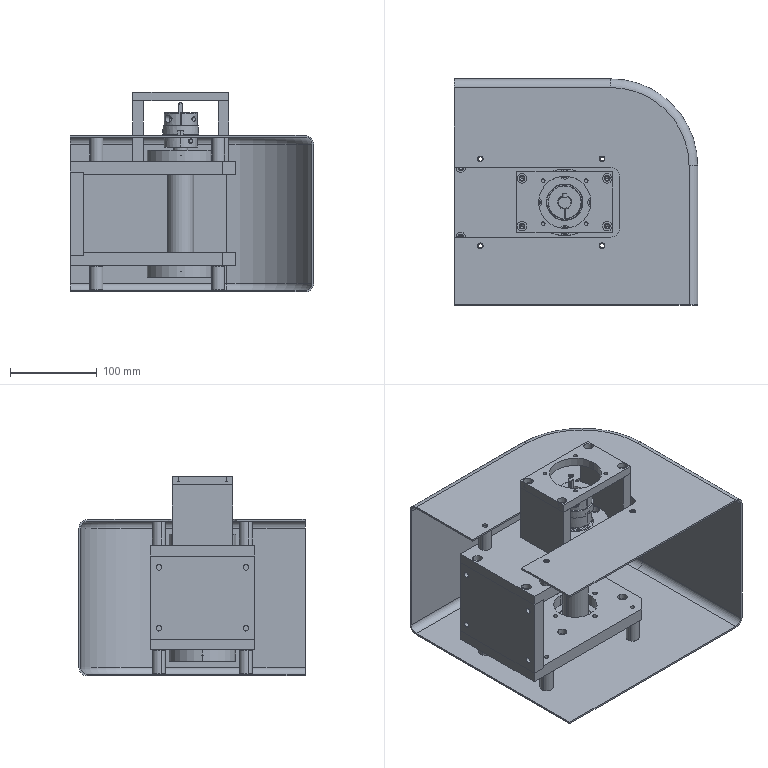Assembly | SolidWorks | mm | 30 component files | 30 solids | 814 faces | box 280 x 260 x 230 mm | volume 1605857 mm3 | cylinder 379 | plane 244 | cone 161 | torus 30 | commonest cylinder face diameters 5 x73 11 x56 6.6 x40 6.5 x32 6.647 x16 15 x16 16 x15 42 x12
Bill of materials:
10X8X50ParallelKey | 1 | AISI 1045 Steel, cold drawn | Flat bar with fully rounded (semicircular) ends, giving an obround outline, with small rounded edges all round.
17x5x5ParallelKey | 1 | AISI 1045 Steel, cold drawn | Thick obround prism (two parallel flat sides, semicircular ends) with chamfered edges on both faces.
25x5x5ParallelKey | 1 | AISI 1045 Steel, cold drawn | Slender obround prism with chamfered perimeter edges. Similar to the previous part but narrower relative to its length.
bearingB6905ZZ | 2 | AISI 1045 Steel, cold drawn | Plain annular ring (flat washer-like cylinder with a central through-bore). The top face shows thin concentric circular lines near the outer and inner edges.
housing_BGRRB6905ZZ | 2 | AISI 1045 Steel, cold drawn | Circular flange disc with a large central bore, four through-holes equally spaced on a bolt circle, and a shorter, smaller-diameter spigot/step on one face.
RRING42 | 2 | AISI 1045 Steel, cold drawn | Thin, flat, split ring with an open gap. Both ends have inward-projecting lugs, each with a small round hole.
M5 | 2 | AISI 1045 Steel, cold drawn | Headed cylindrical pin/screw-like body: a short, larger-diameter cylindrical head with a chamfered outer edge, and a longer smaller-diameter plain cylindrical shank with a chamfered tip.
MCOCG_spacer38 | 1 | AISI 1045 Steel, cold drawn | Thick annular disc with a central through-hole and a straight rectangular slot running across each face. The slots appear to sit at different angular positions, and a small notch is cut at the bore edge.
MCOCGXK3816 | 2 | AISI 1045 Steel, cold drawn | Split-type collar: a cylindrical ring with a central bore that has a rectangular keyway, a narrow radial slit through one side, transverse holes through the body, and a rectangular tab projecting axially from one face.
WT-FLD-EJG-1212-00-019 | 1 | AISI 1045 Steel, cold drawn | Flat rectangular plate with a large central circular through-opening, four larger corner holes, and four smaller holes arranged around the central opening.
WT-FLD-EJG-1212-00-020 | 2 | AISI 1045 Steel, cold drawn | Rectangular block/thick plate with plain large faces. Two round holes are drilled into one narrow edge face near each end.
WT-FLD-EJG-1212-00-006 | 2 | AISI 1045 Steel, cold drawn | Rectangular plate with two chamfered corners at one end. It has a large round through-opening offset toward the chamfered end, surrounded by four small holes at 90 degrees, several additional hole patterns, and a stepped edge (rabbet) on one side.
WT-FLD-EJG-1212-00-007 | 1 | AISI 1045 Steel, cold drawn | Thick rectangular plate block with four through holes near the corners of the large face and two small holes in one narrow edge face.
WT-FLD-EJG-1212-00-008 | 1 | AISI 1045 Steel, cold drawn | Stepped cylindrical shaft with a long main body, reduced-diameter steps at both ends, and a keyway slot on the smallest end journal.
WT-FLD-EJG-1212-00-023 | 1 | AISI 1045 Steel, cold drawn | Thin bent sheet part with a C-shaped cross-section: a top flange and a bottom flange joined by a vertical wall that wraps around one large-radius rounded corner in plan view.
WT-FLD-EJG-1212-00-024 | 8 | AISI 1045 Steel, cold drawn | Plain cylindrical tube or spacer with a central through bore and chamfered outer end edges.
Mates:
1. coincident | WT-FLD-EJG-1212-00-006-1 face at (-127, 0, 48) dir (0, 0, -1) | WT-FLD-EJG-1212-00-007-1 face at (-112, -60, 48) dir (0, 0, 1)
2. coincident | WT-FLD-EJG-1212-00-006-1 face at (-127, 0, 60) dir (0, 0, 1) | BGRRB6905ZZ-1/housing_BGRRB6905ZZ-1 face at (0, 0, 60) dir (0, 0, -1)
3. concentric | WT-FLD-EJG-1212-00-006-1 face at (0, 0, 45) dir (0, 0, 1) r 25 | BGRRB6905ZZ-1/housing_BGRRB6905ZZ-1 face at (0, 0, 60) dir (0, 0, -1) r 25
4. coincident | WT-FLD-EJG-1212-00-008-1 face at (0, 10, -25) dir (0, 1, 0) | 10X8X50ParallelKey-1 face at (0, 10, -25) dir (0, -1, 0)
5. concentric | WT-FLD-EJG-1212-00-008-1 face at (0, 15, 25) dir (0, -1, 0) r 5 | 10X8X50ParallelKey-1 face at (0, 10, 25) dir (0, 1, 0) r 5
6. concentric | WT-FLD-EJG-1212-00-008-1 face at (0, 15, -25) dir (0, -1, 0) r 5 | 10X8X50ParallelKey-1 face at (0, 10, -25) dir (0, 1, 0) r 5
7. concentric | WT-FLD-EJG-1212-00-008-1 face at (0, 0, -70) dir (0, 0, -1) r 15 | assembly face at (0, 0, 132) dir (0, 0, -1) r 8
8. parallel | WT-FLD-EJG-1212-00-006-1 face at (63, 60, 45) dir (0, 1, 0) | ServoDriveMotorModule-1/WT-FLD-EJG-1212-00-019-1 face at (-55, 35, 140) dir (0, 1, 0)
9. coincident | WT-FLD-EJG-1212-00-006-1 face at (-127, 0, 60) dir (0, 0, 1) | ServoDriveMotorModule-1/WT-FLD-EJG-1212-00-020-1 face at (-49, 0, 60) dir (0, 0, -1)
10. coincident | WT-FLD-EJG-1212-00-008-1 face at (0, 5, 75) dir (0, 1, 0) | 17x5x5ParallelKey-1 face at (0, 5, 87) dir (0, -1, 0)
11. concentric | WT-FLD-EJG-1212-00-008-1 face at (0, 15, 75) dir (0, -1, 0) r 2.5 | 17x5x5ParallelKey-1 face at (0, 10, 75) dir (0, -1, 0) r 2.5
12. coincident | WT-FLD-EJG-1212-00-008-1 face at (2.5, 15, 75) dir (-1, 0, 0) | 17x5x5ParallelKey-1 face at (2.5, 10, 87) dir (1, 0, 0)
13. coincident | assembly face at (2.5, 5, 103) dir (0, 1, 0) | 25x5x5ParallelKey-1 face at (0, 5, 105.5) dir (0, -1, 0)
14. concentric | assembly face at (0, 5.693, 125.5) dir (0, 1, 0) r 2.5 | 25x5x5ParallelKey-1 face at (0, 5, 125.5) dir (0, 1, 0) r 2.5
15. coincident | assembly face at (2.5, 7.599, 103) dir (-1, 0, 0) | 25x5x5ParallelKey-1 face at (2.5, 5, 105.5) dir (1, 0, 0)
16. parallel | WT-FLD-EJG-1212-00-006-1 plane at (-127, 0, 60) dir (1, 0, 0) | BGRRB6905ZZ-1 plane at (0, 0, 58) dir (-1, 0, 0)
17. concentric | WT-FLD-EJG-1212-00-006-1 face at (-119.5, 40, 60) dir (0, 0, 1) r 3.3 | WT-FLD-EJG-1212-00-007-1 face at (-119.5, 40, 48) dir (0, 0, 1) r 2.5
18. concentric | WT-FLD-EJG-1212-00-006-1 face at (-119.5, -40, 60) dir (0, 0, 1) r 3.3 | WT-FLD-EJG-1212-00-007-1 face at (-119.5, -40, 48) dir (0, 0, 1) r 2.5
19. coincident | WT-FLD-EJG-1212-00-007-1 face at (-127, 0, 0) dir (-1, 0, 0) | WT-FLD-EJG-1212-00-023-1 face at (-127, -118, -90) dir (-1, 0, 0)
20. coincident | WT-FLD-EJG-1212-00-023-1 plane at (-127, -118, 0) dir (0, 0, -1) | assembly plane at (0, 0, 0) dir (0, 0, 1)
21. distance | WT-FLD-EJG-1212-00-006-2 face at (63, 60, -45) dir (0, 1, 0) | WT-FLD-EJG-1212-00-023-1 face at (-127, 140, -90) dir (0, -1, 0)
22. coincident | WT-FLD-EJG-1212-00-006-1 face at (-127, 0, 60) dir (0, 0, 1) | WT-FLD-EJG-1212-00-024-1 face at (-97, -50, 60) dir (0, 0, -1)
23. concentric | WT-FLD-EJG-1212-00-006-1 face at (-97, -50, 60) dir (0, 0, 1) r 2.5 | WT-FLD-EJG-1212-00-024-1 face at (-97, -50, 60) dir (0, 0, -1) r 3.25
24. distance | bearingB6905ZZ-1 plane at (2, 0, 0) dir (1, 0, 0) | housing_BGRRB6905ZZ-1 plane at (2, 0, 0) dir (1, 0, 0)
25. coincident | housing_BGRRB6905ZZ-1 axis at (80.9, 0, 0) dir (-1, 0, 0) | bearingB6905ZZ-1 axis at (82.9, 0, 0) dir (-1, 0, 0)
26. coincident | housing_BGRRB6905ZZ-1 axis at (80.9, 0, 0) dir (-1, 0, 0) | bearingB6905ZZ-1 axis at (82.9, 0, 0) dir (-1, 0, 0)
27. coincident | housing_BGRRB6905ZZ-1 axis at (80.9, 0, 0) dir (-1, 0, 0) | bearingB6905ZZ-1 axis at (82.9, 0, 0) dir (-1, 0, 0)
28. angle | bearingB6905ZZ-1 plane at (2, 0, 0) dir (0, 0, -1) | housing_BGRRB6905ZZ-1 plane at (0, 0, 0) dir (0, 0, -1)
29. coincident | WT-FLD-EJG-1212-00-019-1 face at (0, 0, 2) dir (0, 0, 1) | WT-FLD-EJG-1212-00-020-1 face at (49, 0, 2) dir (0, 0, -1)
30. concentric | WT-FLD-EJG-1212-00-019-1 face at (49, 27.5, -8) dir (0, 0, -1) r 5.5 | WT-FLD-EJG-1212-00-020-1 face at (49, 27.5, 2) dir (0, 0, -1) r 2.5
31. concentric | WT-FLD-EJG-1212-00-019-1 face at (49, -27.5, -8) dir (0, 0, -1) r 3.3 | WT-FLD-EJG-1212-00-020-1 face at (49, -27.5, 2) dir (0, 0, -1) r 2.5